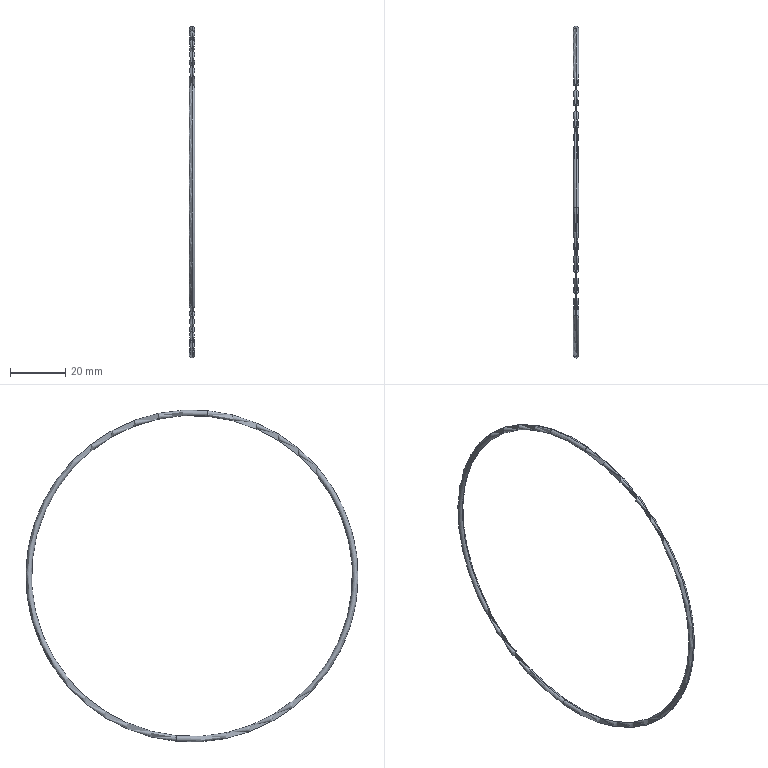Component | SolidWorks | 6O-ring-1 | 1 solid | 4 faces | box 2 x 120 x 120 mm | volume 1165 mm3 | torus 4
build123d program:
from build123d import *

# Parameters (mm, degrees)
SWEEP1_PROFILE_R = 1


with BuildPart() as part:
    # Sweep1: sweep along a path in Sketch8
    with BuildLine(Plane.XY) as sweep1_path:
        CenterArc((0, 0), 59, 0, 360)
    # Sweep1 profile (on start of the path) → Sweep1 (sweep)
    with BuildSketch(Plane(origin=(59, 0, 0), x_dir=(0, 0, 1), z_dir=(0, 1, 0))):
        Circle(SWEEP1_PROFILE_R)
    sweep(path=sweep1_path.line)


solid = part.part

# Placed as in the assembly
solid = solid.moved(Location((-145.89, -90.191, 512), (0, 90, 0)))
STEP:
#1=CARTESIAN_POINT('',(-5.744,-3.325,17.806));
#2=VERTEX_POINT('',#1);
#3=CARTESIAN_POINT('',(-5.744,-3.332,17.885));
#4=VERTEX_POINT('',#3);
#5=CARTESIAN_POINT('',(-5.744,-3.328,17.845));
#6=DIRECTION('',(0.,0.9954,0.09577));
#7=DIRECTION('',(0.,-0.09577,0.9954));
#8=AXIS2_PLACEMENT_3D('',#5,#6,#7);
#9=CIRCLE('',#8,0.03937);
#10=EDGE_CURVE('',#2,#4,#9,.T.);
#11=ORIENTED_EDGE('',*,*,#10,.F.);
#12=CARTESIAN_POINT('',(-5.744,-3.777,22.509));
#13=VERTEX_POINT('',#12);
#14=CARTESIAN_POINT('',(-5.744,-3.551,20.157));
#15=DIRECTION('',(-1.,0.,-0.));
#16=DIRECTION('',(0.,0.,1.));
#17=AXIS2_PLACEMENT_3D('',#14,#15,#16);
#18=CIRCLE('',#17,2.362);
#19=EDGE_CURVE('',#2,#13,#18,.T.);
#20=ORIENTED_EDGE('',*,*,#19,.T.);
#21=CARTESIAN_POINT('',(-5.744,-3.77,22.43));
#22=VERTEX_POINT('',#21);
#23=CARTESIAN_POINT('',(-5.744,-3.773,22.47));
#24=DIRECTION('',(-0.,-0.9954,-0.09577));
#25=DIRECTION('',(0.,0.09577,-0.9954));
#26=AXIS2_PLACEMENT_3D('',#23,#24,#25);
#27=CIRCLE('',#26,0.03937);
#28=EDGE_CURVE('',#13,#22,#27,.T.);
#29=ORIENTED_EDGE('',*,*,#28,.T.);
#30=CARTESIAN_POINT('',(-5.744,-3.551,20.157));
#31=DIRECTION('',(-1.,0.,-0.));
#32=DIRECTION('',(0.,0.,1.));
#33=AXIS2_PLACEMENT_3D('',#30,#31,#32);
#34=CIRCLE('',#33,2.283);
#35=EDGE_CURVE('',#4,#22,#34,.T.);
#36=ORIENTED_EDGE('',*,*,#35,.F.);
#37=EDGE_LOOP('',(#11,#20,#29,#36));
#38=FACE_OUTER_BOUND('',#37,.T.);
#39=CARTESIAN_POINT('',(-5.744,-3.551,20.157));
#40=DIRECTION('',(-1.,0.,-0.));
#41=DIRECTION('',(-0.,-0.09577,0.9954));
#42=AXIS2_PLACEMENT_3D('',#39,#40,#41);
#43=TOROIDAL_SURFACE('',#42,2.323,0.03937);
#44=ADVANCED_FACE('',(#38),#43,.T.);
#45=ORIENTED_EDGE('',*,*,#28,.F.);
#46=CARTESIAN_POINT('',(-5.744,-3.551,20.157));
#47=DIRECTION('',(-1.,0.,-0.));
#48=DIRECTION('',(0.,0.,1.));
#49=AXIS2_PLACEMENT_3D('',#46,#47,#48);
#50=CIRCLE('',#49,2.362);
#51=EDGE_CURVE('',#13,#2,#50,.T.);
#52=ORIENTED_EDGE('',*,*,#51,.T.);
#53=ORIENTED_EDGE('',*,*,#10,.T.);
#54=CARTESIAN_POINT('',(-5.744,-3.551,20.157));
#55=DIRECTION('',(-1.,0.,-0.));
#56=DIRECTION('',(0.,0.,1.));
#57=AXIS2_PLACEMENT_3D('',#54,#55,#56);
#58=CIRCLE('',#57,2.283);
#59=EDGE_CURVE('',#22,#4,#58,.T.);
#60=ORIENTED_EDGE('',*,*,#59,.F.);
#61=EDGE_LOOP('',(#45,#52,#53,#60));
#62=FACE_OUTER_BOUND('',#61,.T.);
#63=CARTESIAN_POINT('',(-5.744,-3.551,20.157));
#64=DIRECTION('',(-1.,0.,-0.));
#65=DIRECTION('',(-0.,-0.09577,0.9954));
#66=AXIS2_PLACEMENT_3D('',#63,#64,#65);
#67=TOROIDAL_SURFACE('',#66,2.323,0.03937);
#68=ADVANCED_FACE('',(#62),#67,.T.);
#69=ORIENTED_EDGE('',*,*,#51,.F.);
#70=CARTESIAN_POINT('',(-5.744,-3.773,22.47));
#71=DIRECTION('',(-0.,-0.9954,-0.09577));
#72=DIRECTION('',(0.,0.09577,-0.9954));
#73=AXIS2_PLACEMENT_3D('',#70,#71,#72);
#74=CIRCLE('',#73,0.03937);
#75=EDGE_CURVE('',#22,#13,#74,.T.);
#76=ORIENTED_EDGE('',*,*,#75,.F.);
#77=ORIENTED_EDGE('',*,*,#59,.T.);
#78=CARTESIAN_POINT('',(-5.744,-3.328,17.845));
#79=DIRECTION('',(0.,0.9954,0.09577));
#80=DIRECTION('',(0.,-0.09577,0.9954));
#81=AXIS2_PLACEMENT_3D('',#78,#79,#80);
#82=CIRCLE('',#81,0.03937);
#83=EDGE_CURVE('',#4,#2,#82,.T.);
#84=ORIENTED_EDGE('',*,*,#83,.T.);
#85=EDGE_LOOP('',(#69,#76,#77,#84));
#86=FACE_OUTER_BOUND('',#85,.T.);
#87=CARTESIAN_POINT('',(-5.744,-3.551,20.157));
#88=DIRECTION('',(-1.,0.,-0.));
#89=DIRECTION('',(-0.,-0.09577,0.9954));
#90=AXIS2_PLACEMENT_3D('',#87,#88,#89);
#91=TOROIDAL_SURFACE('',#90,2.323,0.03937);
#92=ADVANCED_FACE('',(#86),#91,.T.);
#93=ORIENTED_EDGE('',*,*,#19,.F.);
#94=ORIENTED_EDGE('',*,*,#83,.F.);
#95=ORIENTED_EDGE('',*,*,#35,.T.);
#96=ORIENTED_EDGE('',*,*,#75,.T.);
#97=EDGE_LOOP('',(#93,#94,#95,#96));
#98=FACE_OUTER_BOUND('',#97,.T.);
#99=CARTESIAN_POINT('',(-5.744,-3.551,20.157));
#100=DIRECTION('',(-1.,0.,-0.));
#101=DIRECTION('',(-0.,-0.09577,0.9954));
#102=AXIS2_PLACEMENT_3D('',#99,#100,#101);
#103=TOROIDAL_SURFACE('',#102,2.323,0.03937);
#104=ADVANCED_FACE('',(#98),#103,.T.);
#105=CLOSED_SHELL('',(#44,#68,#92,#104));
#106=MANIFOLD_SOLID_BREP('',#105);
#107=CARTESIAN_POINT('',(0.,0.,0.));
#108=DIRECTION('',(0.,0.,1.));
#109=DIRECTION('',(1.,0.,0.));
#110=AXIS2_PLACEMENT_3D('',#107,#108,#109);
#111=(LENGTH_UNIT()NAMED_UNIT(*)SI_UNIT($,.METRE.));
#112=LENGTH_MEASURE_WITH_UNIT(LENGTH_MEASURE(0.0254),#111);
#113=DIMENSIONAL_EXPONENTS(1.,0.,0.,0.,0.,0.,0.);
#114=(CONVERSION_BASED_UNIT('',#112)LENGTH_UNIT()NAMED_UNIT(#113));
#115=UNCERTAINTY_MEASURE_WITH_UNIT(LENGTH_MEASURE(0.00001),#114,'','');
#116=(NAMED_UNIT(*)PLANE_ANGLE_UNIT()SI_UNIT($,.RADIAN.));
#117=(NAMED_UNIT(*)SI_UNIT($,.STERADIAN.)SOLID_ANGLE_UNIT());
#118=(GEOMETRIC_REPRESENTATION_CONTEXT(3)GLOBAL_UNCERTAINTY_ASSIGNED_CONTEXT((#115))GLOBAL_UNIT_ASSIGNED_CONTEXT((#114,#116,#117))REPRESENTATION_CONTEXT('',''));
#119=ADVANCED_BREP_SHAPE_REPRESENTATION('',(#106,#110),#118);
#120=COLOUR_RGB('',0.7922,0.8196,0.9333);
#121=FILL_AREA_STYLE_COLOUR('',#120);
#122=FILL_AREA_STYLE('',(#121));
#123=SURFACE_STYLE_FILL_AREA(#122);
#124=SURFACE_SIDE_STYLE('',(#123));
#125=SURFACE_STYLE_USAGE(.BOTH.,#124);
#126=PRESENTATION_STYLE_ASSIGNMENT((#125));
#127=STYLED_ITEM('',(#126),#106);
#128=PRESENTATION_LAYER_ASSIGNMENT('','',(#127));
#129=(LENGTH_UNIT()NAMED_UNIT(*)SI_UNIT($,.METRE.));
#130=LENGTH_MEASURE_WITH_UNIT(LENGTH_MEASURE(0.0254),#129);
#131=DIMENSIONAL_EXPONENTS(1.,0.,0.,0.,0.,0.,0.);
#132=(CONVERSION_BASED_UNIT('',#130)LENGTH_UNIT()NAMED_UNIT(#131));
#133=UNCERTAINTY_MEASURE_WITH_UNIT(LENGTH_MEASURE(0.00001),#132,'','');
#134=(NAMED_UNIT(*)PLANE_ANGLE_UNIT()SI_UNIT($,.RADIAN.));
#135=(NAMED_UNIT(*)SI_UNIT($,.STERADIAN.)SOLID_ANGLE_UNIT());
#136=(GEOMETRIC_REPRESENTATION_CONTEXT(3)GLOBAL_UNCERTAINTY_ASSIGNED_CONTEXT((#133))GLOBAL_UNIT_ASSIGNED_CONTEXT((#132,#134,#135))REPRESENTATION_CONTEXT('',''));
#137=MECHANICAL_DESIGN_GEOMETRIC_PRESENTATION_REPRESENTATION('',(#127),#136);